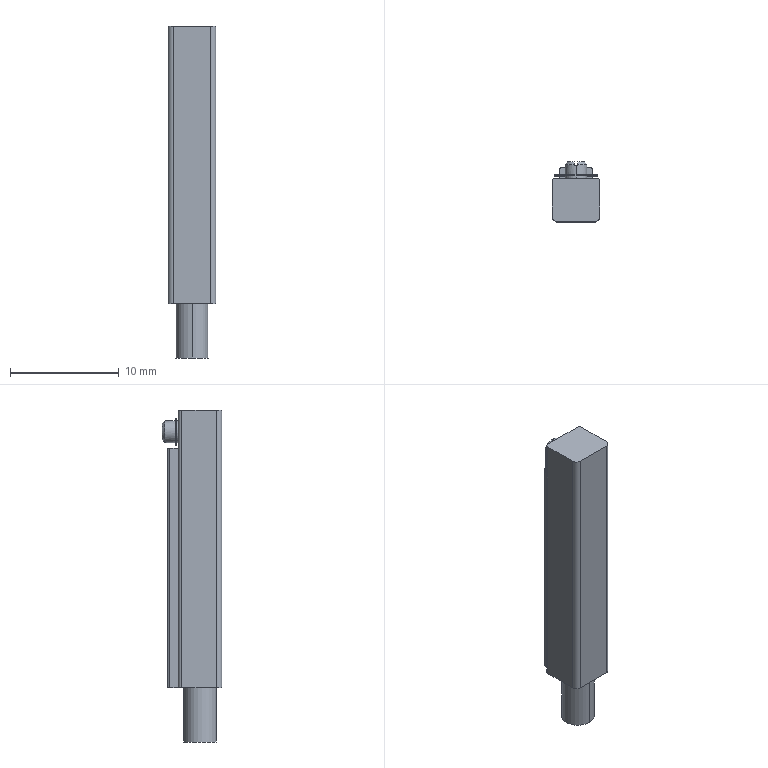Component | SolidWorks | TR-20x75-S-GN-1 (0)-3_6-1 | 1 solid | 45 faces | volume 551 mm3 | plane 27 | cylinder 16 | cone 2 | commonest cylinder face diameters 2 x4 0.5 x4 3 x2 1 x2 0.6 x2 0.4 x2